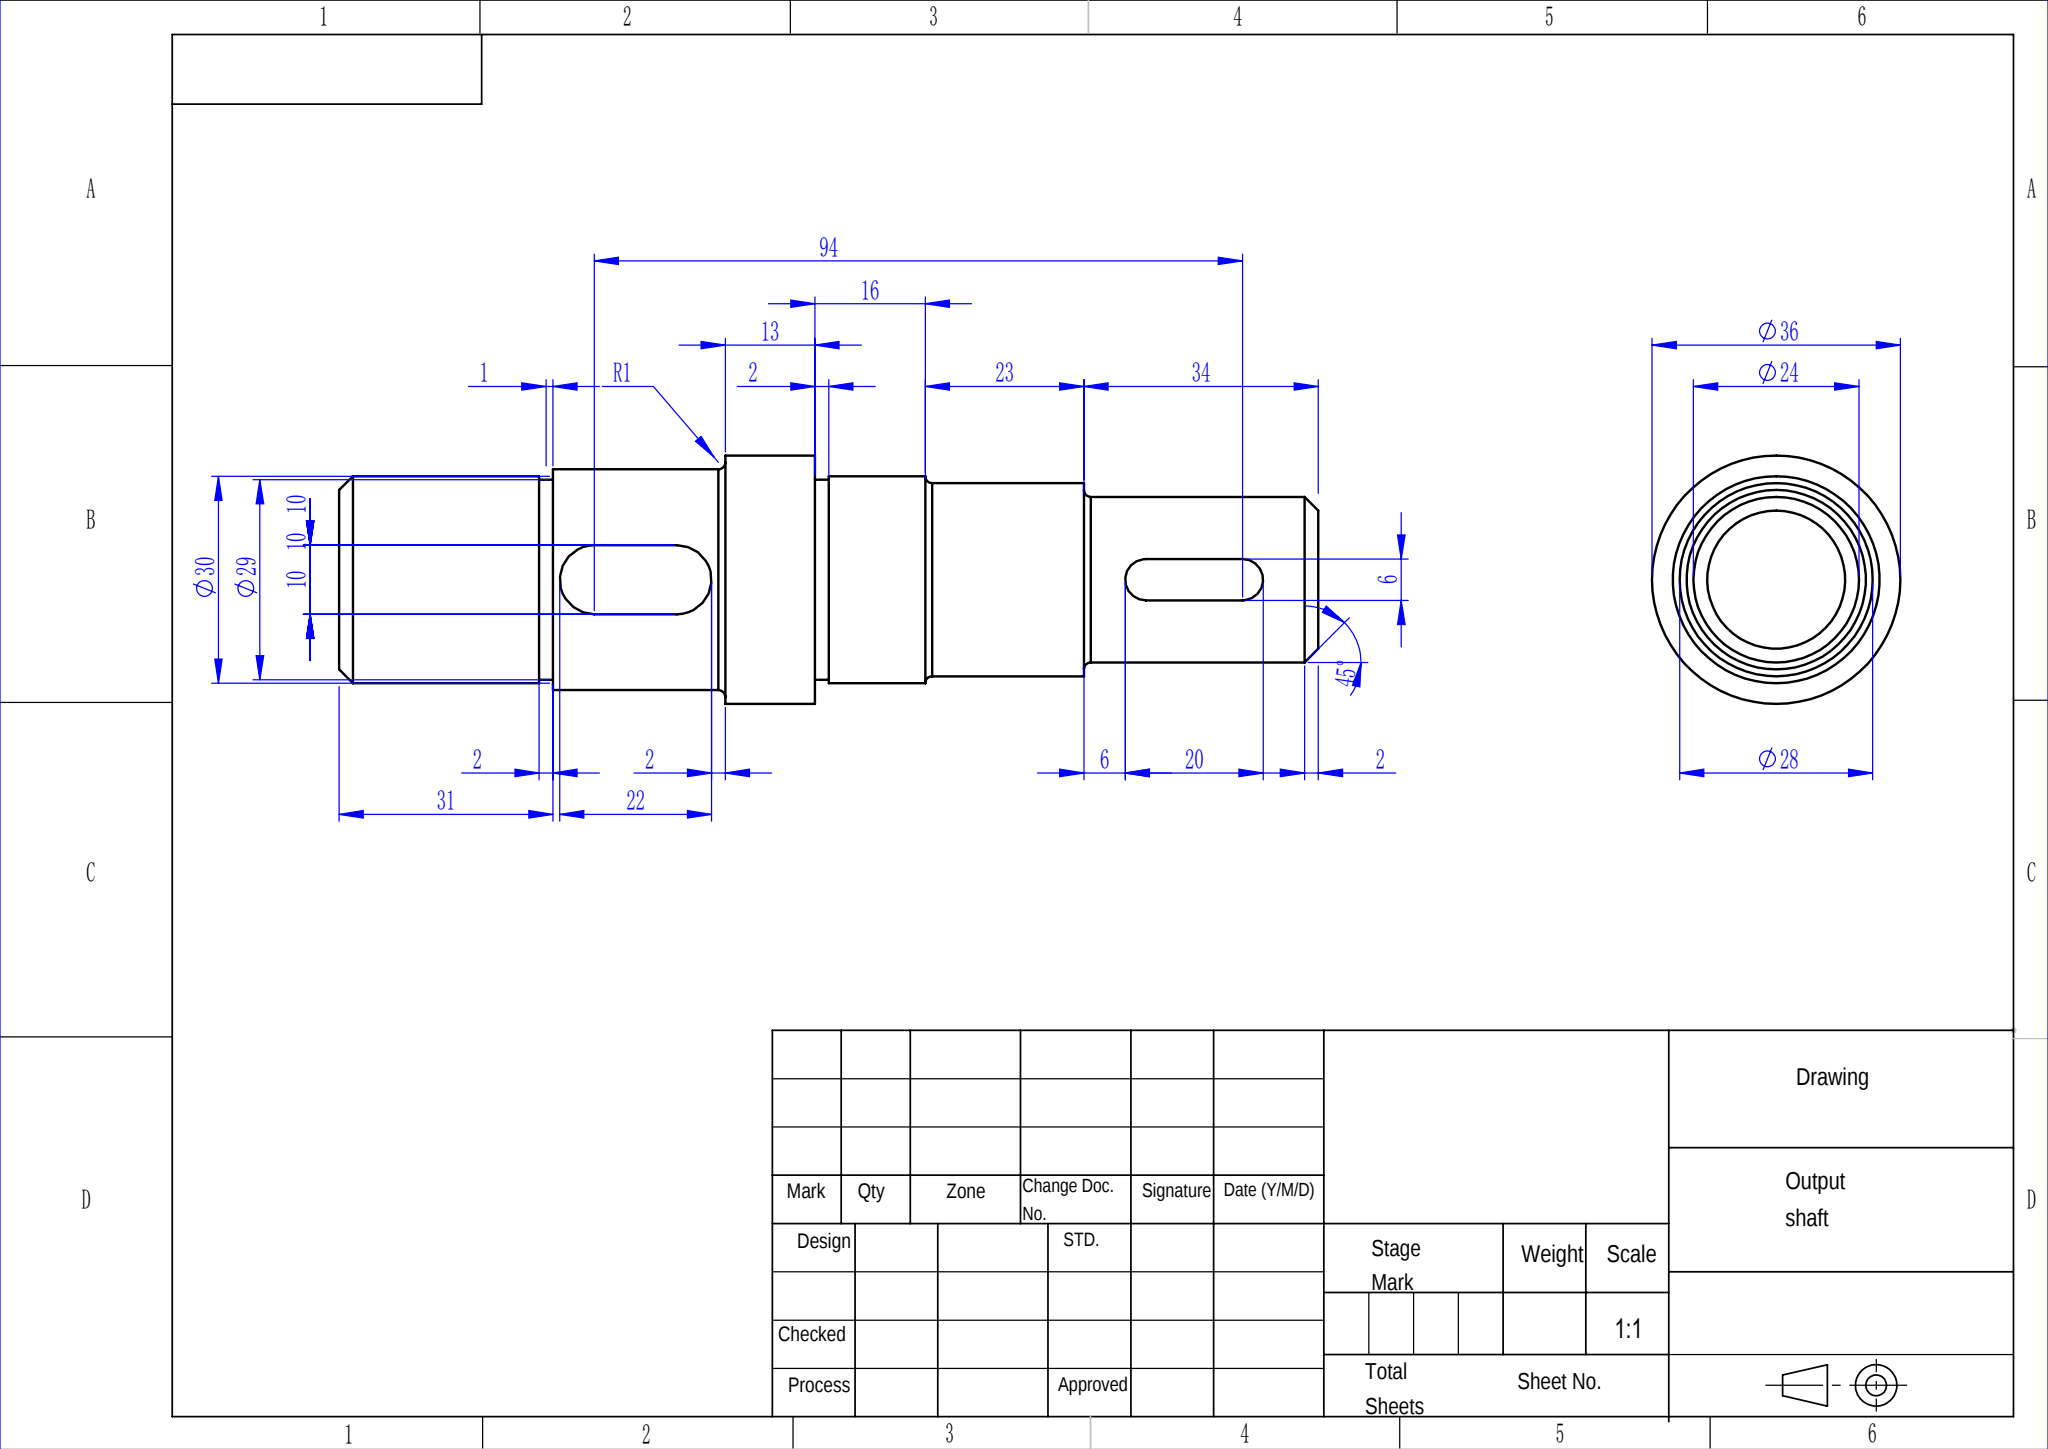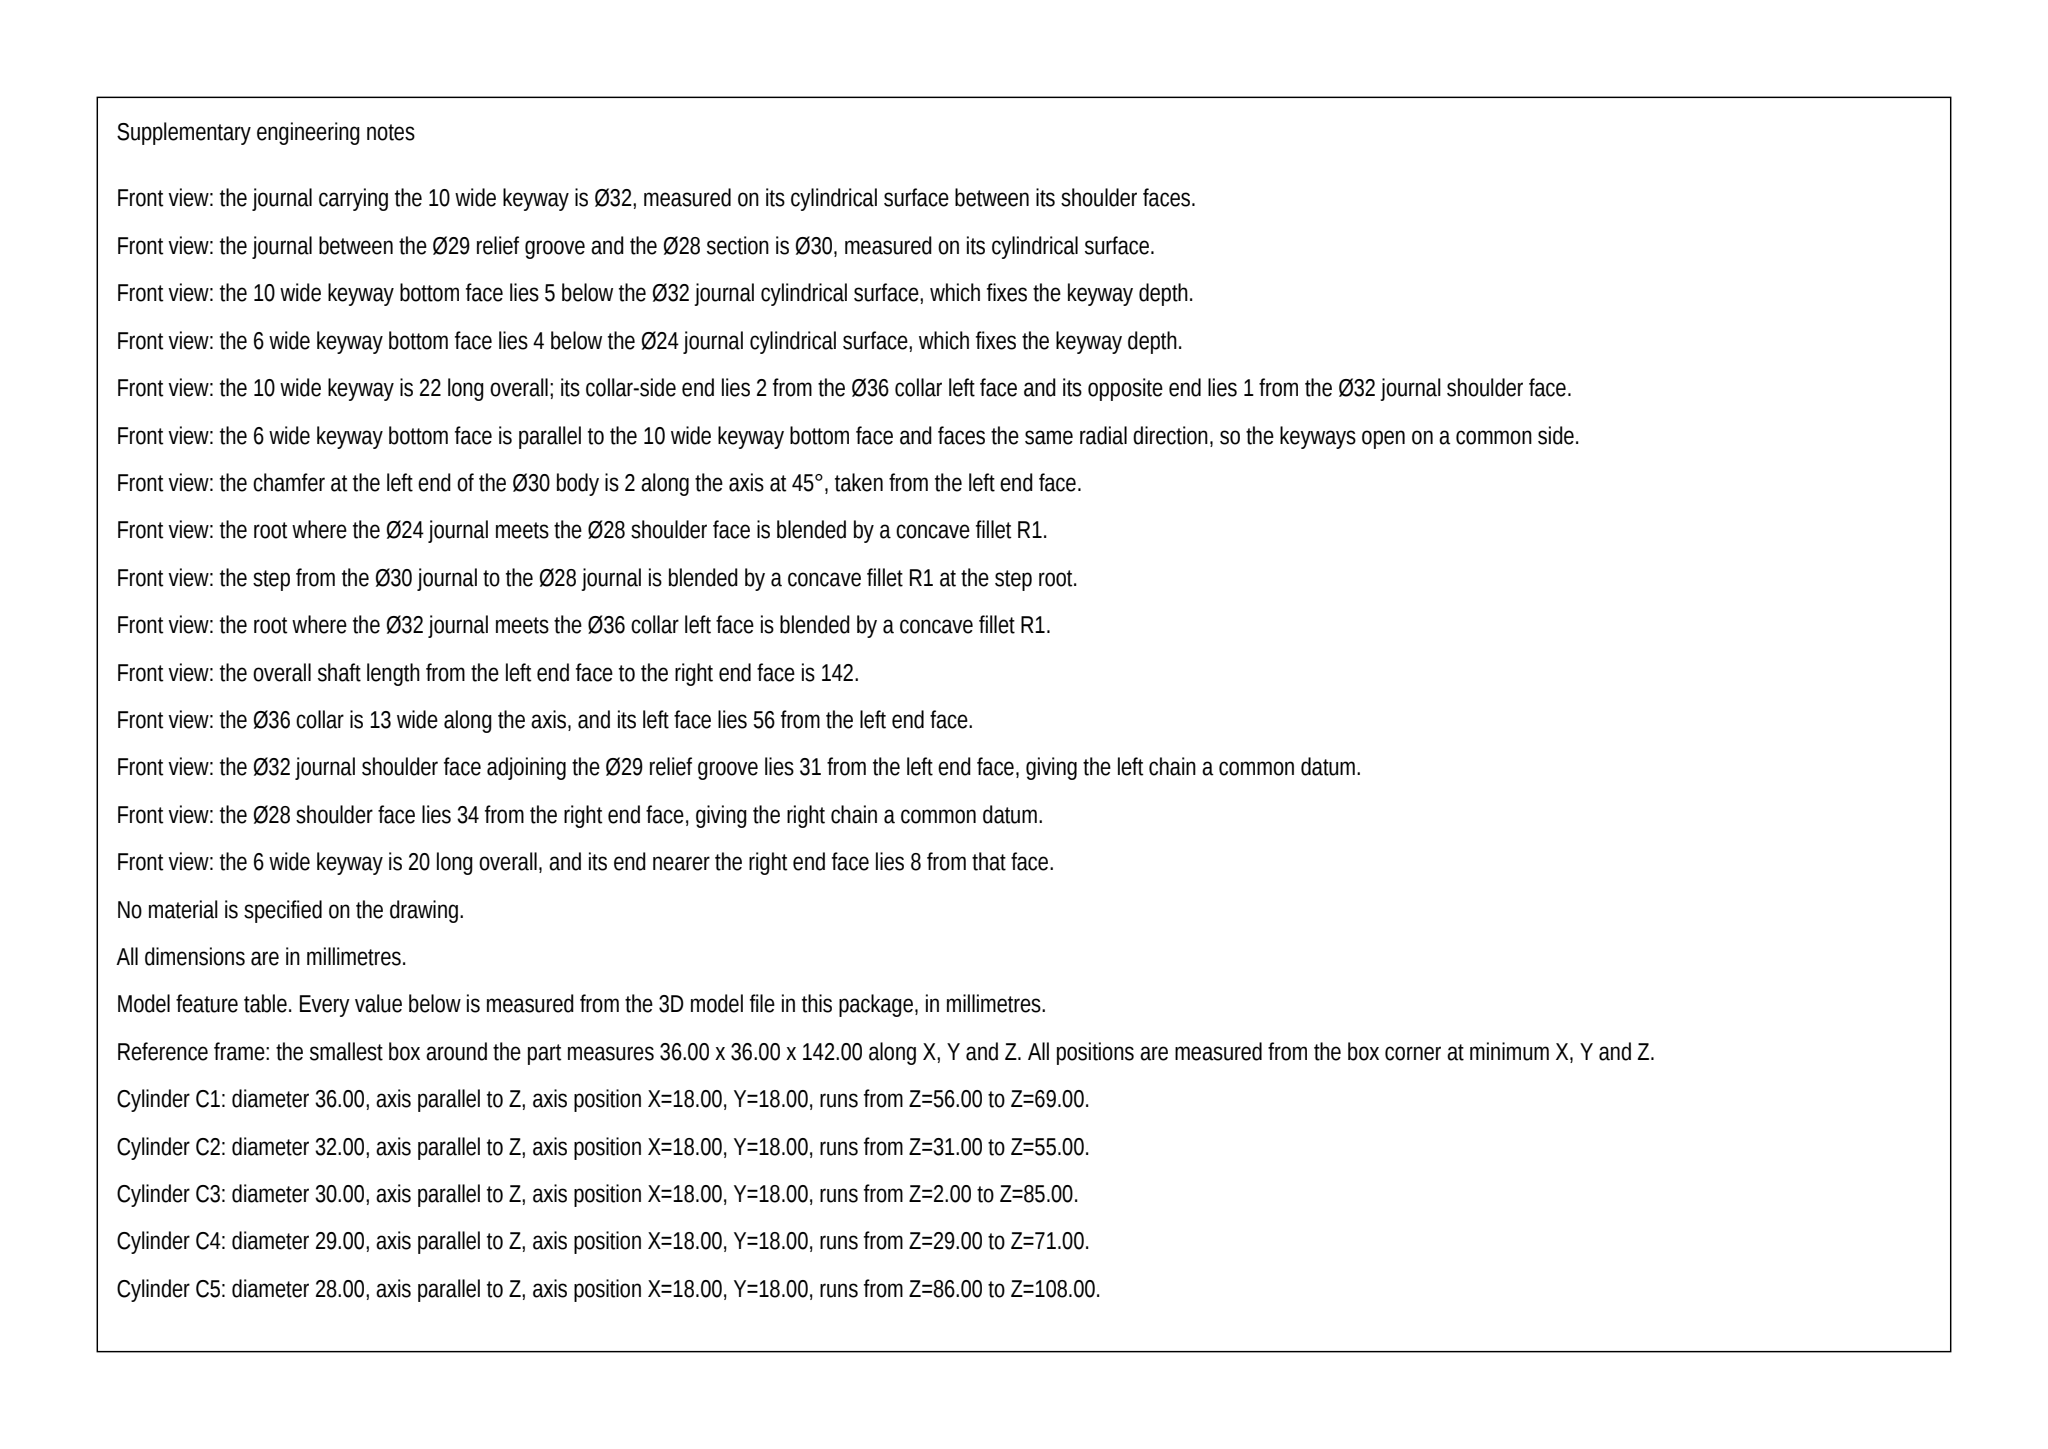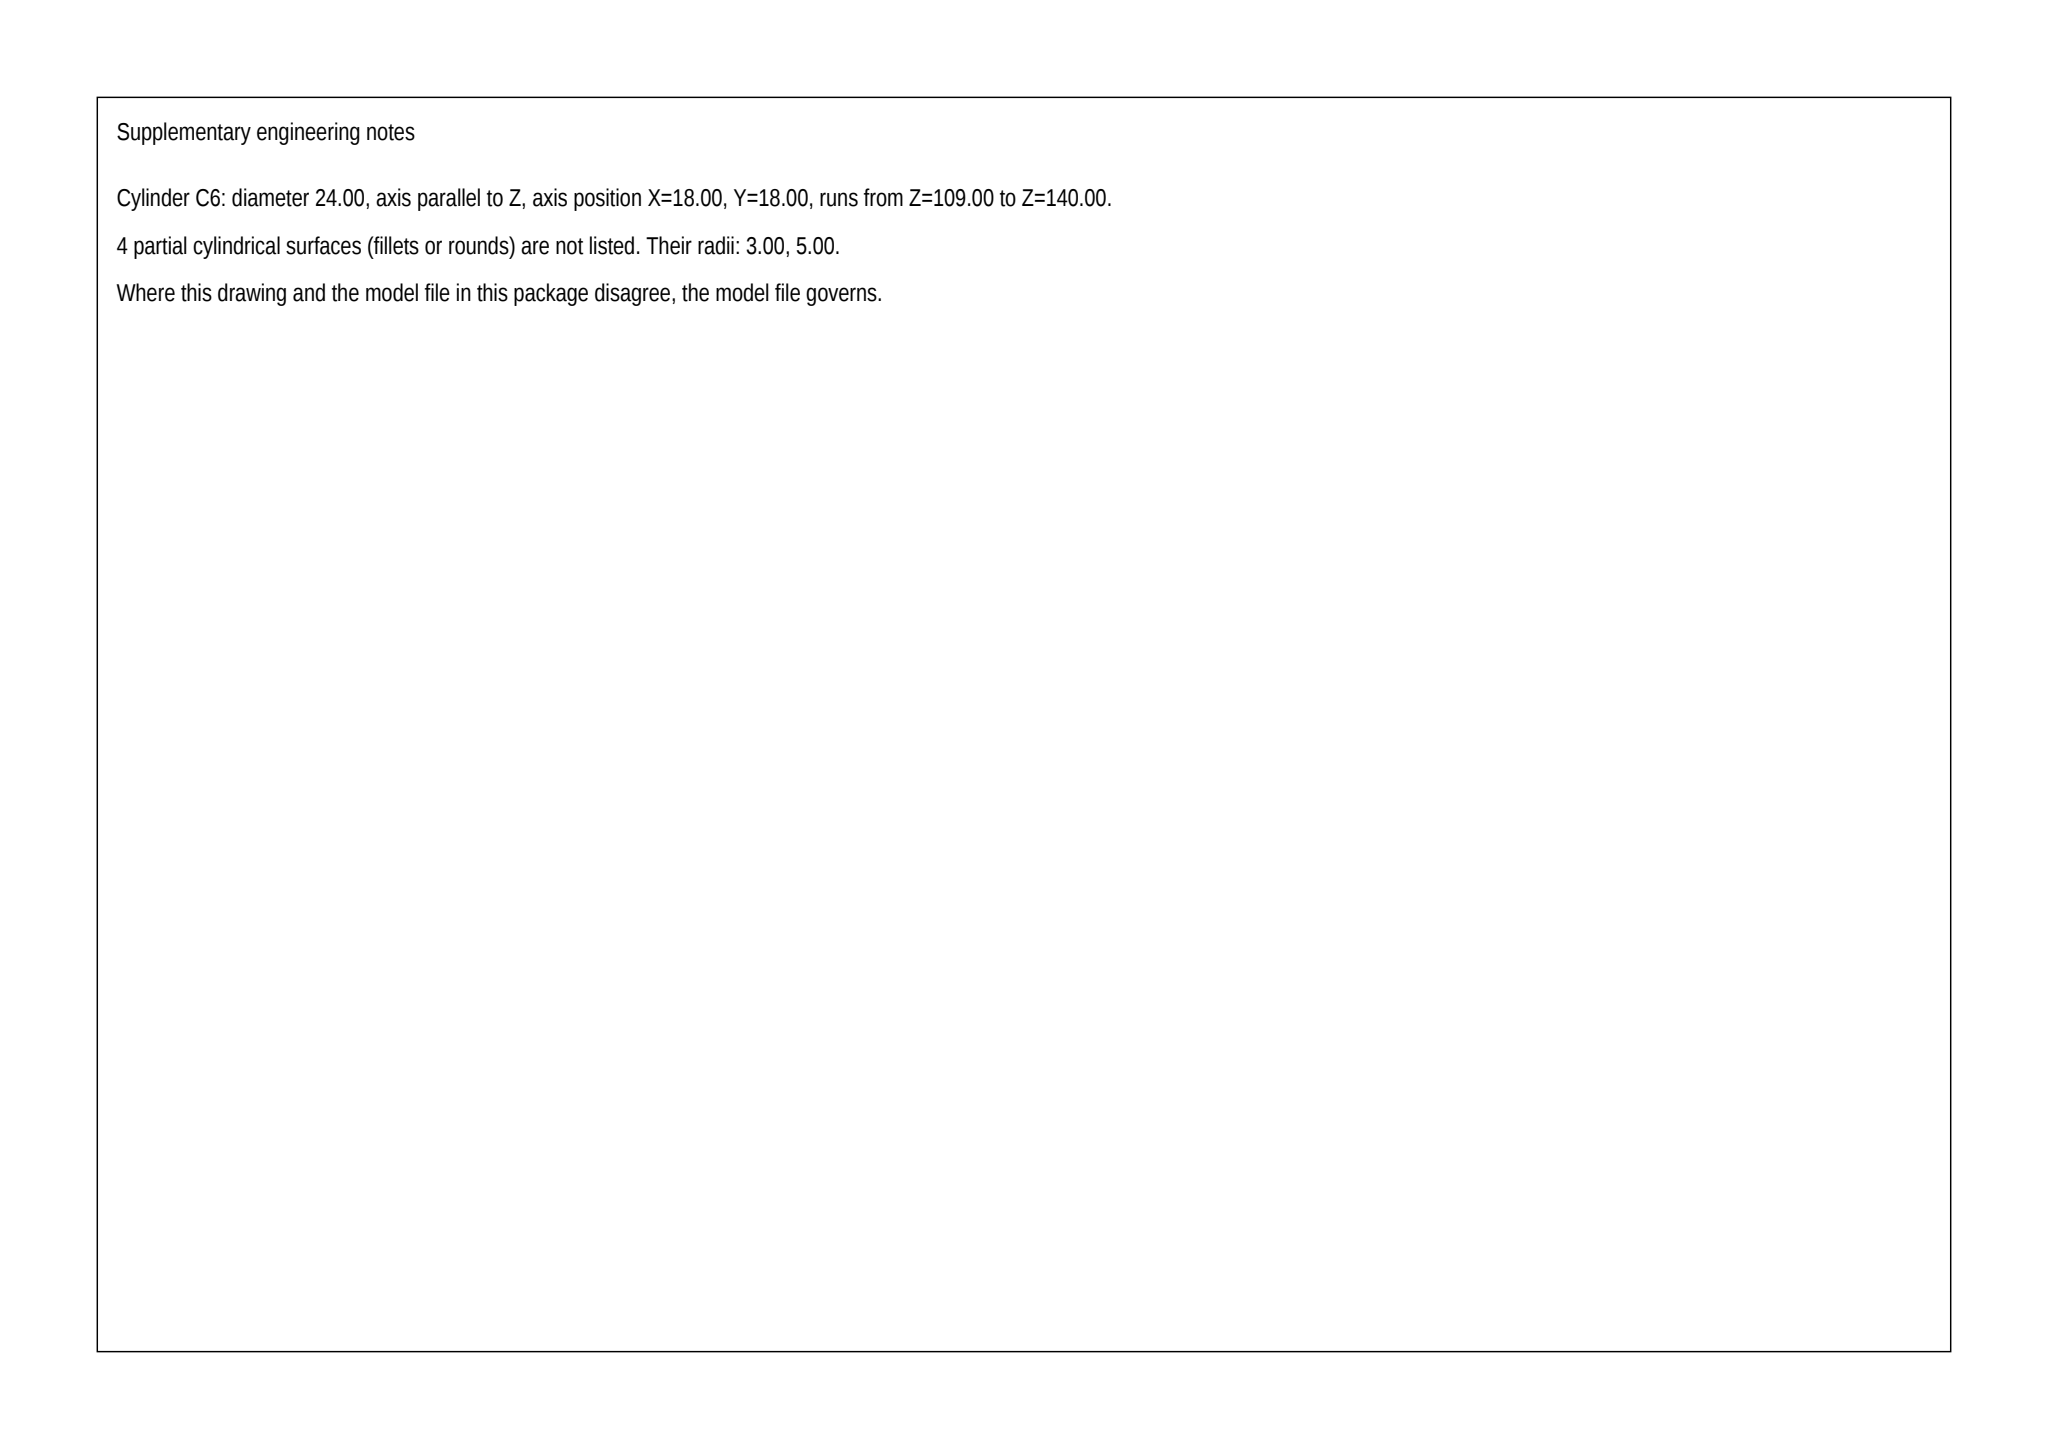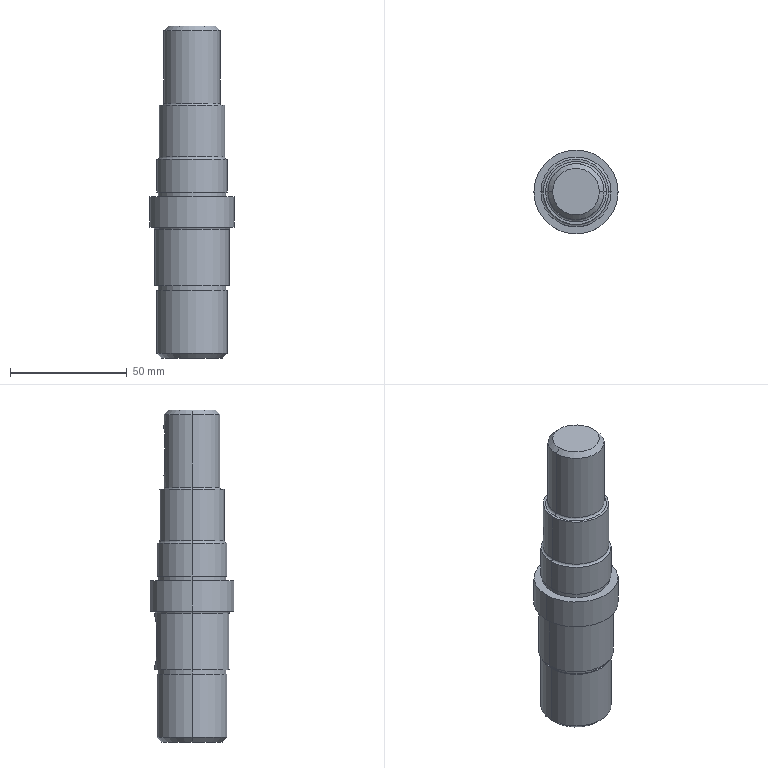Part | SolidWorks | mm | 1 solid | 46 faces | box 36 x 36 x 142 mm | volume 94273 mm3 | cylinder 22 | plane 14 | torus 6 | cone 4 | commonest cylinder face diameters 30 x4 29 x4 6 x3 10 x3 28 x2 36 x2 32 x2 24 x2
Drawing notes:
SLOTTED STEP: Ø32, 24 LONG, FROM 31 TO 55 MM FROM LEFT (Ø30) END FACE | from the solid: cylinders: [32.0,"z",[19.17,19.17,null],24.0] with z-planes at 31 and 56
STEP RIGHT OF Ø36 FLANGE GROOVE: Ø30, 14 LONG, BEGINS 71 MM FROM LEFT END FACE | from the solid: cylinders: [30.0,"z",[19.17,19.17,null],14.0] between z-planes 71 and 108 (with Ø28 x 22)
10 WIDE SLOT ON Ø32 STEP: DEPTH 5 (FLAT FLOOR 11 FROM AXIS), 22 LONG, 31 FROM LEFT END FACE | from the solid: cylinders [10.0,"y",[19.17,null,37.0],5.0] / [10.0,"y",[19.17,null,49.0],5.0] with plane y=30.17 vs axis y=19.17 and Ø32 OD
6 WIDE SLOT ON Ø24 END: DEPTH 4 (FLAT FLOOR 8 FROM AXIS), 20 LONG, 6 FROM Ø28/Ø24 SHOULDER | from the solid: cylinders [6.0,"y",[19.17,null,117.0],4.0] / [6.0,"y",[19.17,null,131.0],4.0] with plane y=27.17 vs axis y=19.17 and Ø24 OD
ALL DIMENSIONS IN MILLIMETERS | from the solid: STEP model units: mm (bbox_xyz 38.338 x 38.338 x 142.0 mm)
CHAMFER AT LEFT (Ø30) END FACE: 2 X 45° (BREAKS Ø30 DOWN TO Ø26), AT 0 MM FROM LEFT END FACE | from the solid: cones[included_angle 90.0, ref_dia 26.0] (90° included = 45° per side, Ø30->Ø26 = 2 mm) at z=0 end of the Ø30 cylinder (dia 30, axis z, length 27, z-plane 0.0)
RELIEF GROOVE RIGHT OF Ø36 FLANGE: Ø29, 2 WIDE, FROM 69 TO 71 MM FROM LEFT (Ø30) END FACE | from the solid: cylinder dia 29.0 about z, length 2.0; axis planes z=69.0 and z=71.0